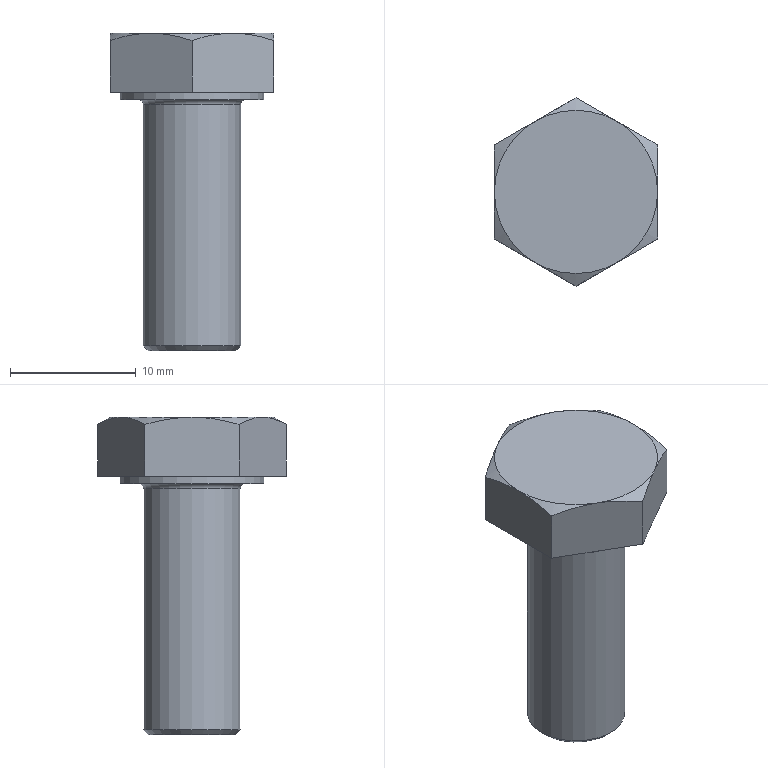Component | NX | GB-T5782-2000_M8X20 | 1 solid | 20 faces | volume 1692 mm3 | plane 10 | cone 7 | cylinder 2 | torus 1 | commonest cylinder face diameters 11.47 x1 7.76 x1